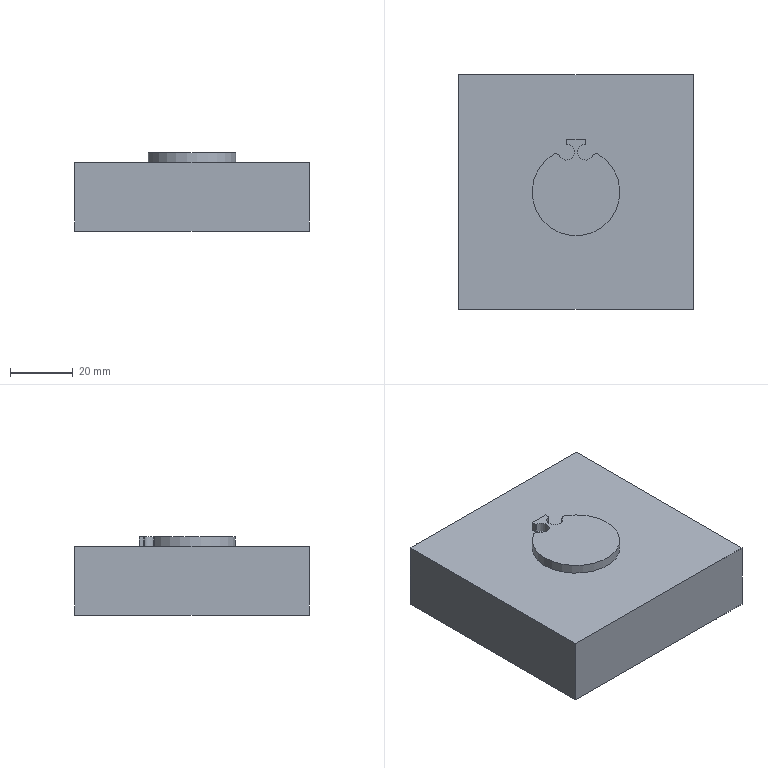CAM job | Mastercam | mm | 7 operations | part box 75 x 75 x 25
1. Facing | 24 - 100 平铣刀
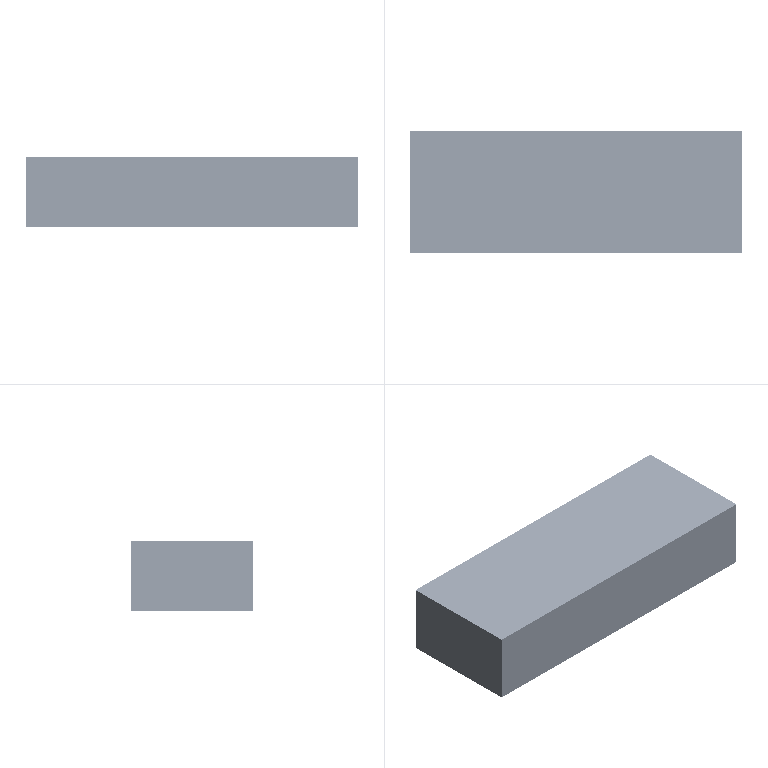2. 2D High Speed (2D Area Mill) | 10 - 10 平铣刀
3. Contour (Remachining) | 4 - 4 平铣刀
4. 2D High Speed (2D Area Mill) | 4 - 4 平铣刀
5. Contour (2D) | 4 - 4 平铣刀
6. Contour (2D chamfer) | 7 - 4 倒角刀
7. Drill/Counterbore | 7 - 4 倒角刀